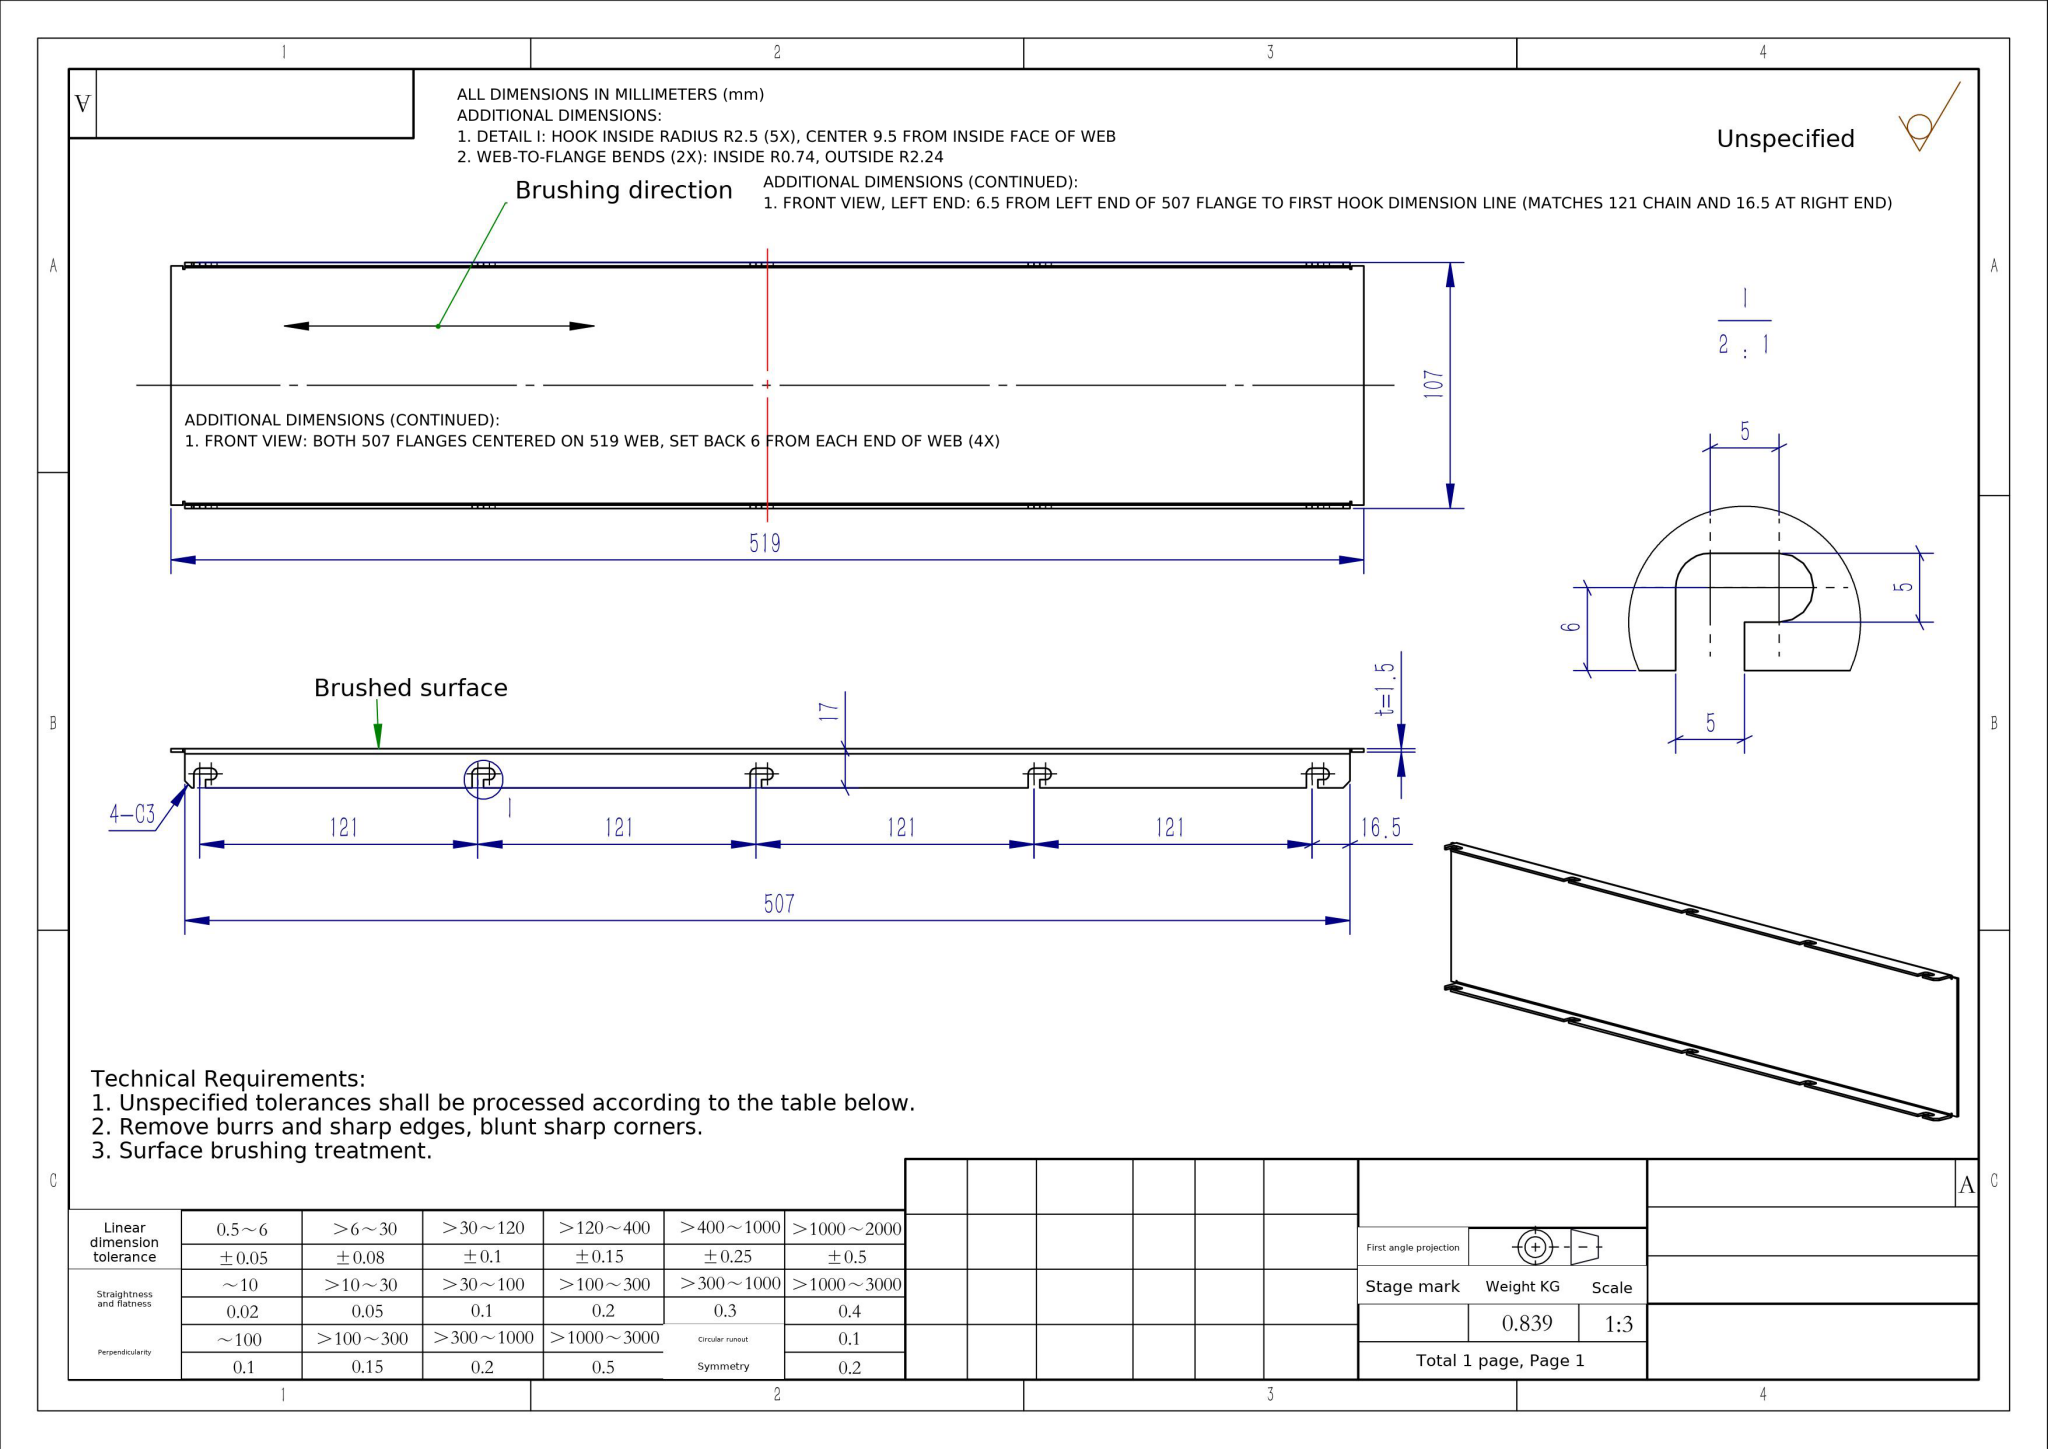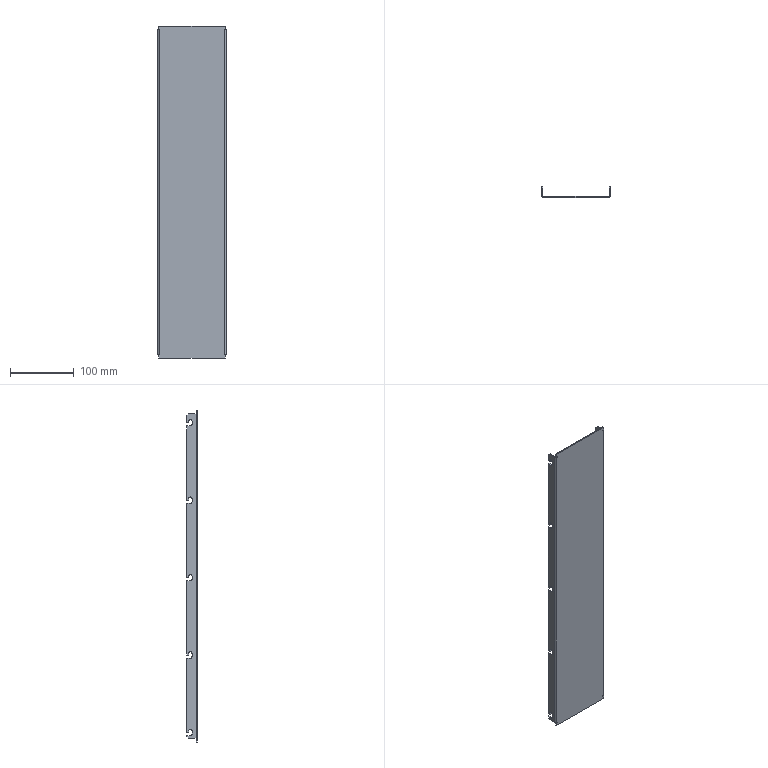Part | NX | mm | 1 solid | 122 faces | box 107 x 17 x 519 mm | volume 104865 mm3 | plane 88 | cylinder 34 | commonest cylinder face diameters 5 x30 4.473 x2 1.473 x2